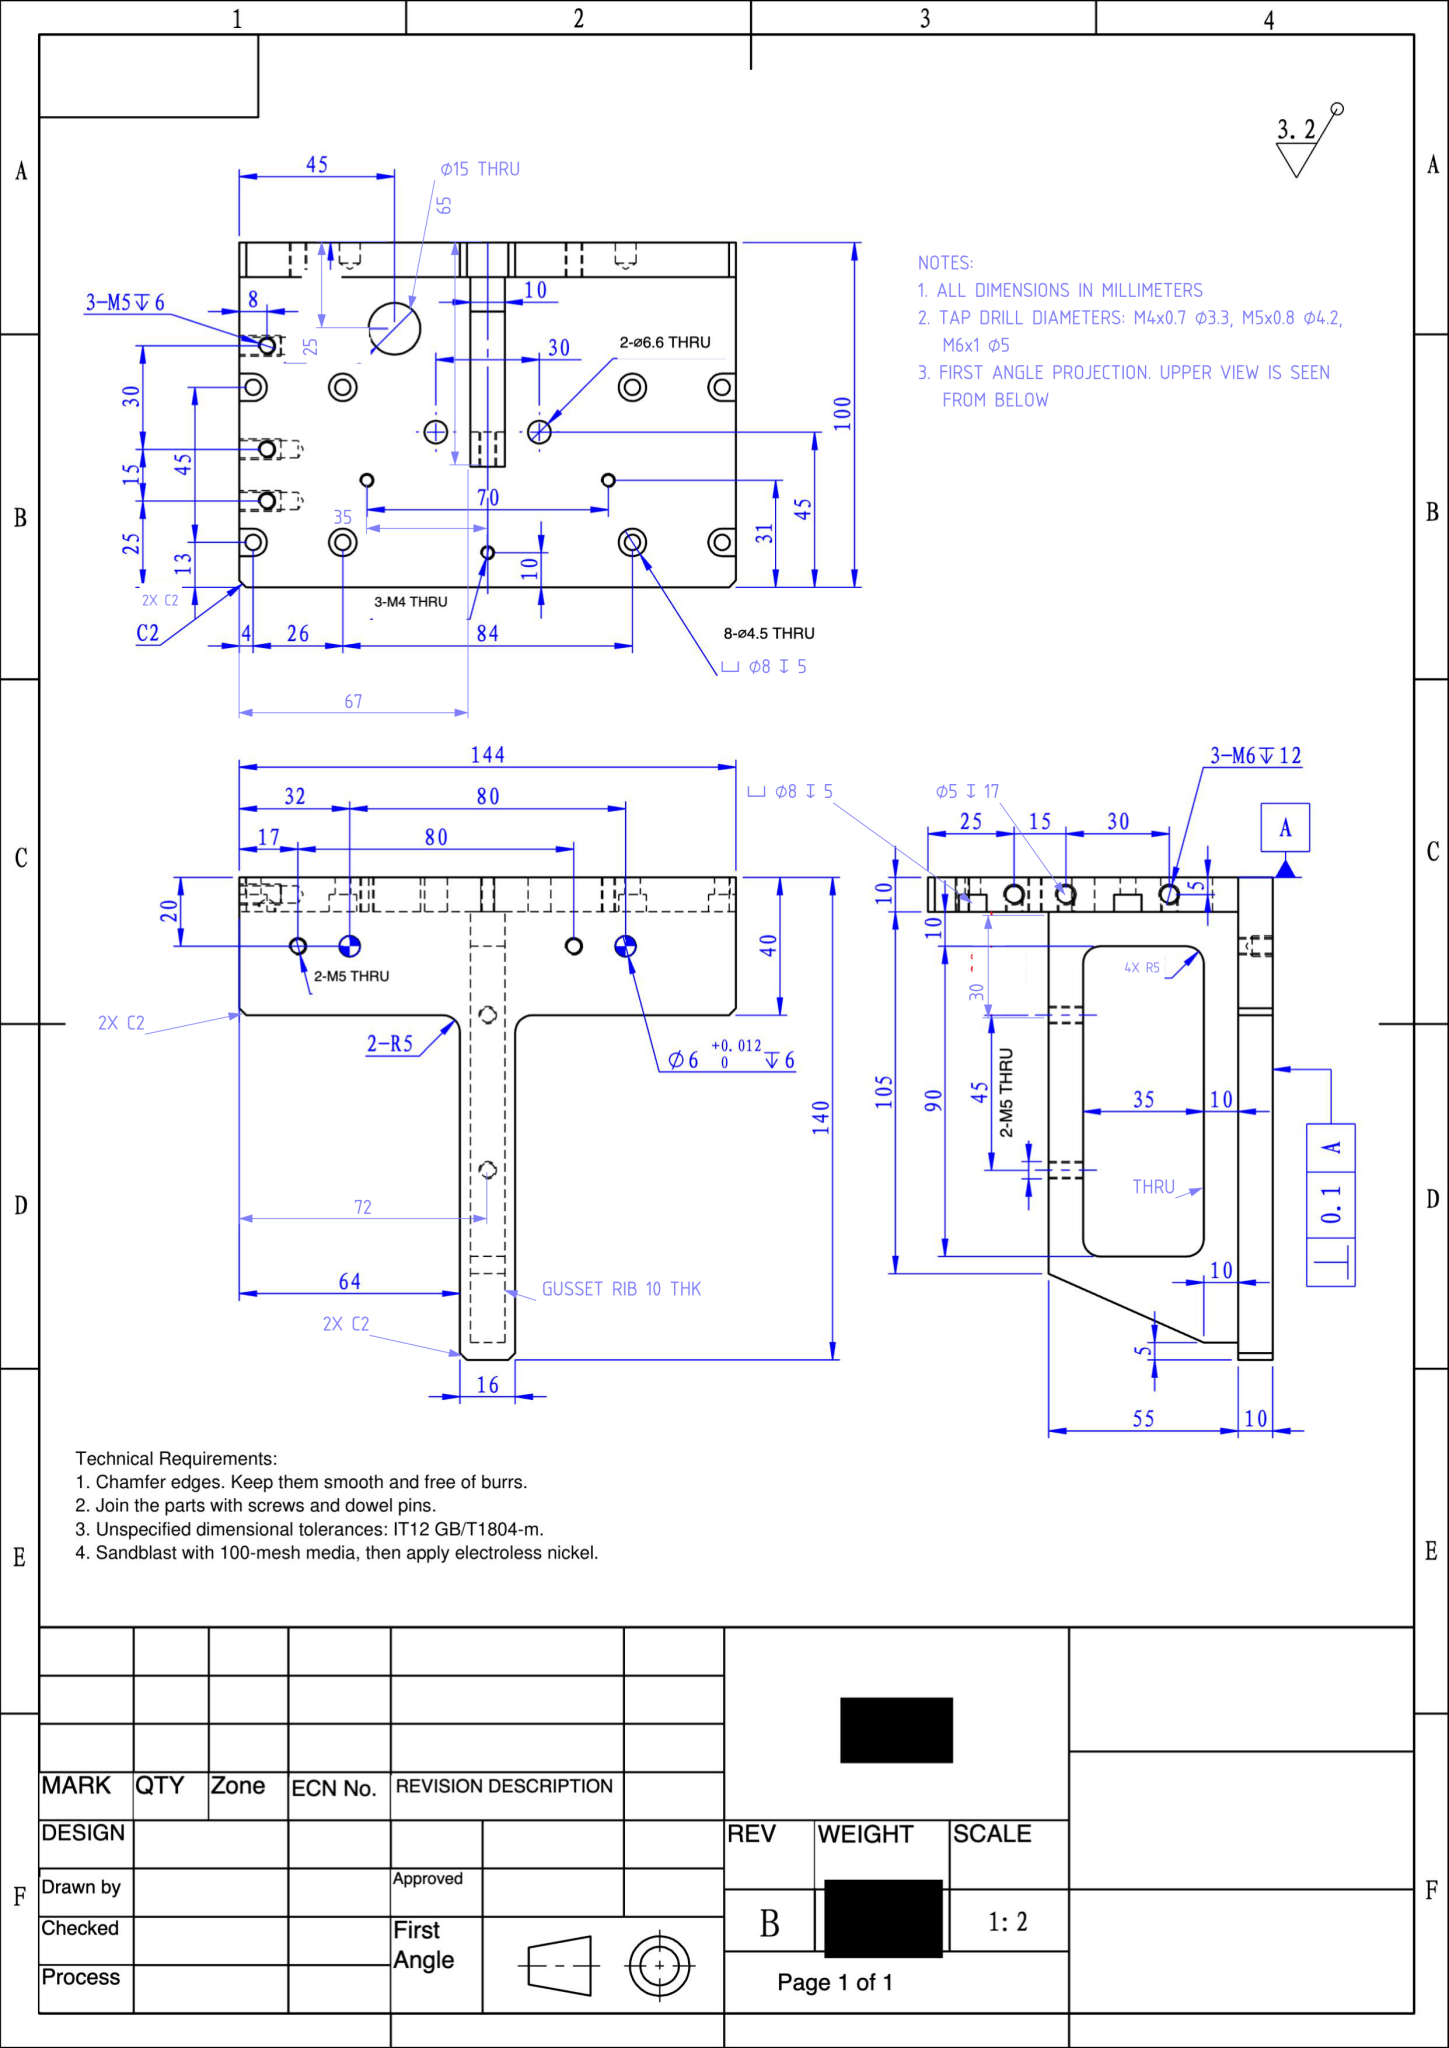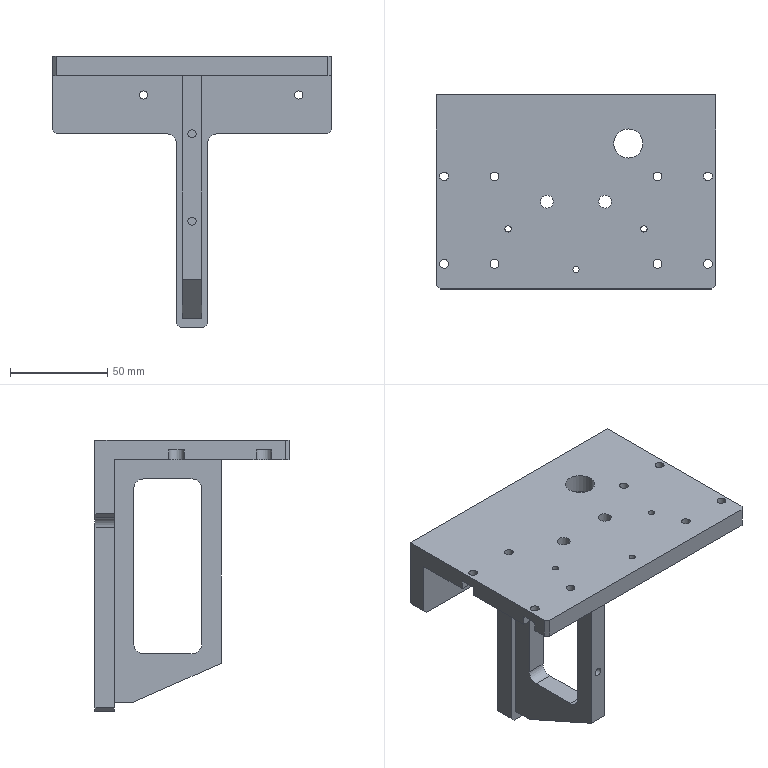Part | NX | mm | 1 solid | 88 faces | box 144 x 100 x 140 mm | volume 228587 mm3 | plane 43 | cylinder 40 | cone 5 | commonest cylinder face diameters 8 x8 4.5 x8 4.2 x7 10 x6 3.3 x3 5 x3 6.6 x2 6 x2